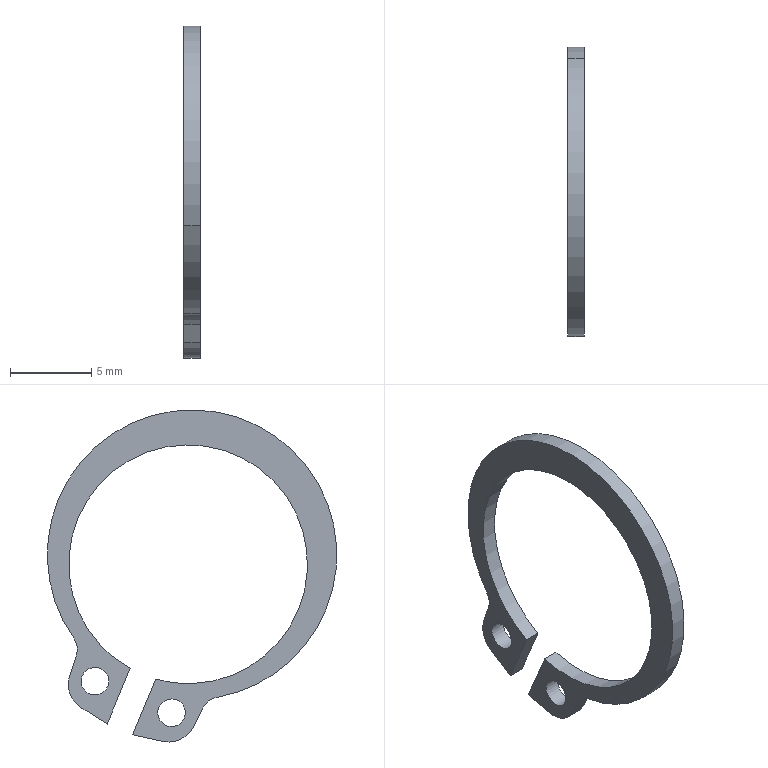Component | NX | CIRCLIP_SHAFT_A16_2 | 1 solid | 22 faces | volume 92 mm3 | cylinder 14 | plane 8 | commonest cylinder face diameters 1.7 x4 14.7 x3 17.825 x3 3.4 x2 2.467 x2